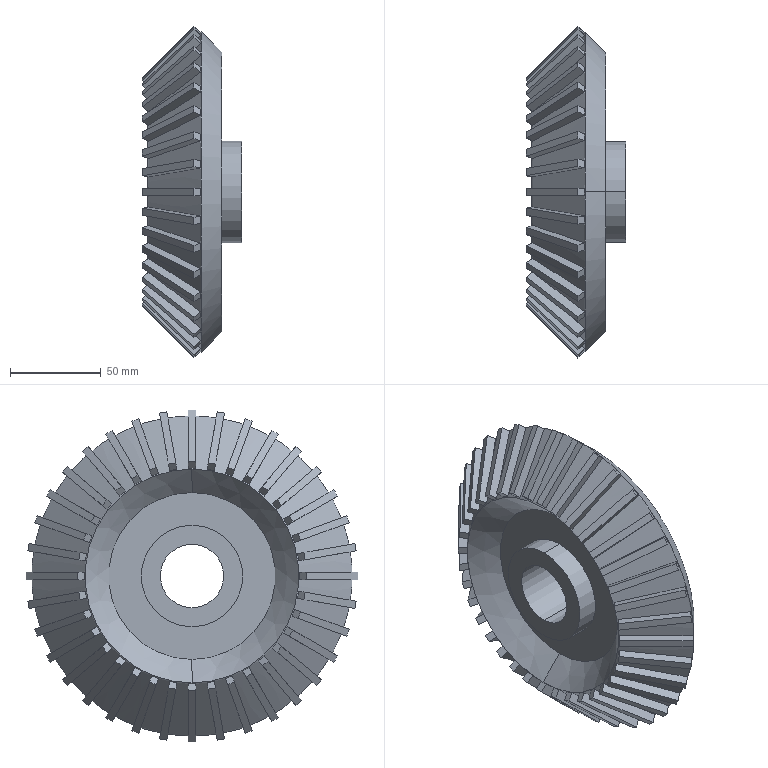Component | SolidWorks | BevelGear-2 | 1 solid | 200 faces | box 54.93 x 183.21 x 183.21 mm | volume 459660 mm3 | plane 184 | cone 10 | cylinder 6 | commonest cylinder face diameters 56 x4 35 x2
build123d program:
from build123d import *

# Parameters (mm, degrees)
SKETCH2_2_W         = 40.39
SKETCH2_2_H         = 4
BOSS_EXTRUDE1_DEPTH = 5
CIRPATTERN5_COUNT   = 36
CHAMFER1_SIZE       = 1.5


with BuildPart() as part:
    # Sketch1_2 → Revolve1 (revolve)
    with BuildSketch(Plane(origin=(0, 0, 0), x_dir=(0, 0, -1), z_dir=(1, 0, 0)), mode=Mode.PRIVATE) as revolve1_sk:
        Polygon((39, 28), (39, 46.093), (51.907, 58.999), (22.441, 88.465), (11.128, 77.151), (29, 59.279), (29, 28), (0, 28), (0, 17.5), (51, 17.5), (51, 28), align=None)
    revolve(revolve1_sk.sketch.rotate(Axis((0, 0, 0), (0, 0, -1)), 90), axis=Axis((0, 0, 0), (0, 0, -1)))

    # Sketch2_2 → Boss-Extrude1 (add, symmetric)
    with BuildSketch(Plane(origin=(55.453, 0, -55.453), x_dir=(-0.7071, 0, -0.7071), z_dir=(0.7071, 0, -0.7071))):
        with Locations((-25.93, 0)):
            Rectangle(SKETCH2_2_W, SKETCH2_2_H)
    boss_extrude1 = extrude(amount=BOSS_EXTRUDE1_DEPTH, both=True)

    # CirPattern5: Boss-Extrude1 ×36 about axis
    cirpattern5_axis = Axis((0, 0, 0), (0, 0, 1))
    for i in range(1, CIRPATTERN5_COUNT):
        add(boss_extrude1.rotate(cirpattern5_axis, i * 360 / CIRPATTERN5_COUNT))

    # Chamfer1
    chamfer1_edges = [part.edges().sort_by_distance(p)[0] for p in [
        (-17.5, 0, 0),
    ]]
    chamfer(chamfer1_edges, length=CHAMFER1_SIZE)


solid = part.part

# Placed as in the assembly
solid = solid.moved(Location((150.528, 15.31, -110), (0, 90, 0)))